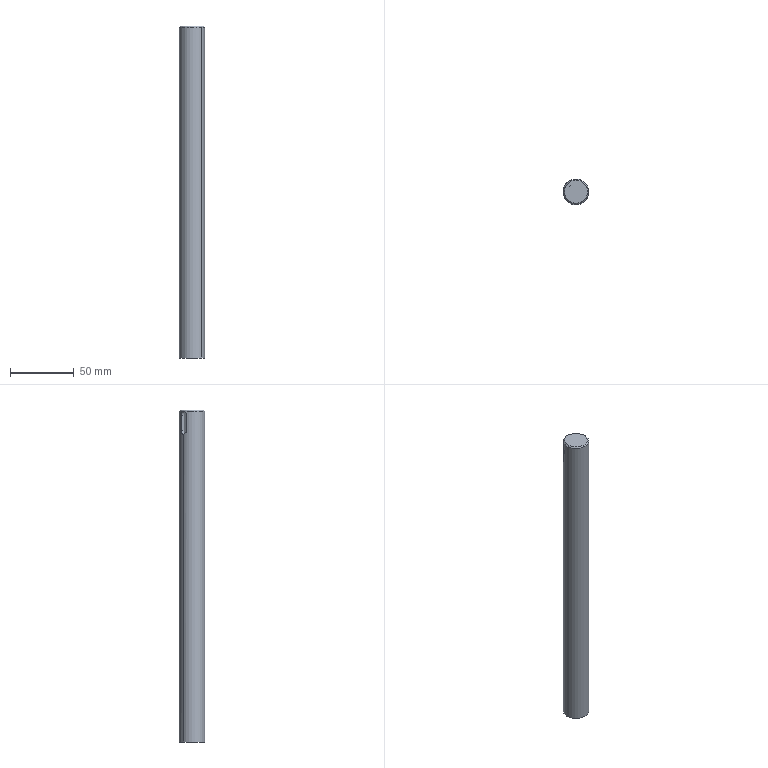Component | SolidWorks | DriveShaft-1 | 1 solid | 11 faces | box 20 x 20 x 260 mm | volume 81314 mm3 | plane 5 | cylinder 4 | cone 2 | commonest cylinder face diameters 20 x2 6 x2
build123d program:
from build123d import *

# Parameters (mm, degrees)
SKETCH1_R           = 10
BOSS_EXTRUDE1_DEPTH = 260
CUT_EXTRUDE1_DEPTH  = 3.5
CHAMFER1_SIZE       = 1


with BuildPart() as part:
    # Sketch1 → Boss-Extrude1 (new body)
    with BuildSketch(Plane(origin=(0, 0, 0), x_dir=(1, 0, 0), z_dir=(0, 1, 0))):
        with Locations(Location((0, 0, 0), (0, 0, 270))):
            Circle(SKETCH1_R)
    extrude(amount=BOSS_EXTRUDE1_DEPTH)

    # Sketch2 → Cut-Extrude1 (cut)
    with BuildSketch(Plane.XY.offset(10)):
        with BuildLine():
            Line((3, 256), (3, 244))
            ThreePointArc((3, 244), (0, 241), (-3, 244))
            Line((-3, 244), (-3, 256))
            ThreePointArc((-3, 256), (0, 259), (3, 256))
        make_face()
    extrude(amount=-CUT_EXTRUDE1_DEPTH, mode=Mode.SUBTRACT)

    # Chamfer1
    chamfer1_edges = [part.edges().sort_by_distance(p)[0] for p in [
        (0, 260, -10),
    ]]
    chamfer(chamfer1_edges, length=CHAMFER1_SIZE)


solid = part.part

# Placed as in the assembly
solid = solid.moved(Location((310.629, 34.1, 218.3), (-90, -48.276, -180)))
STEP:
#1=COLOUR_RGB('',0.7922,0.8196,0.9333);
#2=FILL_AREA_STYLE_COLOUR('',#1);
#3=FILL_AREA_STYLE('',(#2));
#4=SURFACE_STYLE_FILL_AREA(#3);
#5=SURFACE_SIDE_STYLE('',(#4));
#6=SURFACE_STYLE_USAGE(.BOTH.,#5);
#7=PRESENTATION_STYLE_ASSIGNMENT((#6));
#8=CARTESIAN_POINT('',(11.965,1.578,18.831));
#9=VERTEX_POINT('',#8);
#10=CARTESIAN_POINT('',(12.494,1.107,18.831));
#11=VERTEX_POINT('',#10);
#12=CARTESIAN_POINT('',(12.23,1.343,18.831));
#13=DIRECTION('',(0.,0.,1.));
#14=DIRECTION('',(-0.7464,0.6655,0.));
#15=AXIS2_PLACEMENT_3D('',#12,#13,#14);
#16=CIRCLE('',#15,0.3543);
#17=EDGE_CURVE('',#9,#11,#16,.T.);
#18=ORIENTED_EDGE('',*,*,#17,.F.);
#19=CARTESIAN_POINT('',(11.936,1.605,18.791));
#20=VERTEX_POINT('',#19);
#21=CARTESIAN_POINT('',(11.965,1.578,18.831));
#22=DIRECTION('',(-0.5278,0.4706,-0.7071));
#23=VECTOR('',#22,39.37);
#24=LINE('',#21,#23);
#25=EDGE_CURVE('',#9,#20,#24,.T.);
#26=ORIENTED_EDGE('',*,*,#25,.T.);
#27=CARTESIAN_POINT('',(12.523,1.08,18.791));
#28=VERTEX_POINT('',#27);
#29=CARTESIAN_POINT('',(12.23,1.343,18.791));
#30=DIRECTION('',(-0.,-0.,-1.));
#31=DIRECTION('',(-0.7464,0.6655,0.));
#32=AXIS2_PLACEMENT_3D('',#29,#30,#31);
#33=CIRCLE('',#32,0.3937);
#34=EDGE_CURVE('',#28,#20,#33,.T.);
#35=ORIENTED_EDGE('',*,*,#34,.F.);
#36=CARTESIAN_POINT('',(12.494,1.107,18.831));
#37=DIRECTION('',(0.5278,-0.4706,-0.7071));
#38=VECTOR('',#37,39.37);
#39=LINE('',#36,#38);
#40=EDGE_CURVE('',#11,#28,#39,.T.);
#41=ORIENTED_EDGE('',*,*,#40,.F.);
#42=EDGE_LOOP('',(#18,#26,#35,#41));
#43=FACE_OUTER_BOUND('',#42,.T.);
#44=CARTESIAN_POINT('',(12.23,1.343,18.831));
#45=DIRECTION('',(-0.,-0.,-1.));
#46=DIRECTION('',(0.7464,-0.6655,0.));
#47=AXIS2_PLACEMENT_3D('',#44,#45,#46);
#48=CONICAL_SURFACE('',#47,0.3543,0.7854);
#49=ADVANCED_FACE('',(#43),#48,.T.);
#50=CARTESIAN_POINT('',(11.871,1.504,18.201));
#51=VERTEX_POINT('',#50);
#52=CARTESIAN_POINT('',(11.936,1.605,18.083));
#53=VERTEX_POINT('',#52);
#54=CARTESIAN_POINT('',(11.871,1.504,18.201));
#55=CARTESIAN_POINT('',(11.871,1.504,18.193));
#56=CARTESIAN_POINT('',(11.871,1.505,18.185));
#57=CARTESIAN_POINT('',(11.872,1.508,18.17));
#58=CARTESIAN_POINT('',(11.873,1.51,18.163));
#59=CARTESIAN_POINT('',(11.876,1.516,18.148));
#60=CARTESIAN_POINT('',(11.878,1.519,18.141));
#61=CARTESIAN_POINT('',(11.882,1.527,18.129));
#62=CARTESIAN_POINT('',(11.884,1.531,18.123));
#63=CARTESIAN_POINT('',(11.892,1.546,18.106));
#64=CARTESIAN_POINT('',(11.899,1.557,18.098));
#65=CARTESIAN_POINT('',(11.912,1.575,18.089));
#66=CARTESIAN_POINT('',(11.916,1.581,18.086));
#67=CARTESIAN_POINT('',(11.926,1.593,18.083));
#68=CARTESIAN_POINT('',(11.93,1.599,18.083));
#69=CARTESIAN_POINT('',(11.936,1.605,18.083));
#70=B_SPLINE_CURVE_WITH_KNOTS('',3,(#54,#55,#56,#57,#58,#59,#60,#61,#62,#63,#64,#65,#66,#67,#68,#69),.UNSPECIFIED.,.F.,.F.,(4,2,2,2,2,2,2,4),(0.,0.0005898,0.00118,0.001769,0.002359,0.003539,0.004128,0.004718),.UNSPECIFIED.);
#71=EDGE_CURVE('',#51,#53,#70,.T.);
#72=ORIENTED_EDGE('',*,*,#71,.T.);
#73=CARTESIAN_POINT('',(11.936,1.605,8.594));
#74=VERTEX_POINT('',#73);
#75=CARTESIAN_POINT('',(11.936,1.605,18.831));
#76=DIRECTION('',(-0.,-0.,-1.));
#77=VECTOR('',#76,39.37);
#78=LINE('',#75,#77);
#79=EDGE_CURVE('',#53,#74,#78,.T.);
#80=ORIENTED_EDGE('',*,*,#79,.T.);
#81=CARTESIAN_POINT('',(12.523,1.08,8.594));
#82=VERTEX_POINT('',#81);
#83=CARTESIAN_POINT('',(12.23,1.343,8.594));
#84=DIRECTION('',(0.,0.,1.));
#85=DIRECTION('',(-0.7464,0.6655,0.));
#86=AXIS2_PLACEMENT_3D('',#83,#84,#85);
#87=CIRCLE('',#86,0.3937);
#88=EDGE_CURVE('',#74,#82,#87,.T.);
#89=ORIENTED_EDGE('',*,*,#88,.T.);
#90=CARTESIAN_POINT('',(12.523,1.08,18.831));
#91=DIRECTION('',(-0.,-0.,-1.));
#92=VECTOR('',#91,39.37);
#93=LINE('',#90,#92);
#94=EDGE_CURVE('',#28,#82,#93,.T.);
#95=ORIENTED_EDGE('',*,*,#94,.F.);
#96=ORIENTED_EDGE('',*,*,#34,.T.);
#97=CARTESIAN_POINT('',(11.871,1.504,18.673));
#98=VERTEX_POINT('',#97);
#99=CARTESIAN_POINT('',(11.936,1.605,18.791));
#100=CARTESIAN_POINT('',(11.931,1.599,18.791));
#101=CARTESIAN_POINT('',(11.925,1.593,18.791));
#102=CARTESIAN_POINT('',(11.916,1.581,18.788));
#103=CARTESIAN_POINT('',(11.912,1.575,18.785));
#104=CARTESIAN_POINT('',(11.903,1.563,18.779));
#105=CARTESIAN_POINT('',(11.899,1.557,18.776));
#106=CARTESIAN_POINT('',(11.893,1.546,18.767));
#107=CARTESIAN_POINT('',(11.889,1.541,18.762));
#108=CARTESIAN_POINT('',(11.884,1.531,18.751));
#109=CARTESIAN_POINT('',(11.882,1.527,18.745));
#110=CARTESIAN_POINT('',(11.878,1.519,18.733));
#111=CARTESIAN_POINT('',(11.876,1.516,18.726));
#112=CARTESIAN_POINT('',(11.873,1.51,18.712));
#113=CARTESIAN_POINT('',(11.872,1.508,18.704));
#114=CARTESIAN_POINT('',(11.871,1.505,18.689));
#115=CARTESIAN_POINT('',(11.871,1.504,18.681));
#116=CARTESIAN_POINT('',(11.871,1.504,18.673));
#117=B_SPLINE_CURVE_WITH_KNOTS('',3,(#99,#100,#101,#102,#103,#104,#105,#106,#107,#108,#109,#110,#111,#112,#113,#114,#115,#116),.UNSPECIFIED.,.F.,.F.,(4,2,2,2,2,2,2,2,4),(0.004718,0.005307,0.005896,0.006485,0.007074,0.007663,0.008252,0.008842,0.009431),.UNSPECIFIED.);
#118=EDGE_CURVE('',#20,#98,#117,.T.);
#119=ORIENTED_EDGE('',*,*,#118,.T.);
#120=CARTESIAN_POINT('',(11.871,1.504,18.831));
#121=DIRECTION('',(-0.,-0.,-1.));
#122=VECTOR('',#121,39.37);
#123=LINE('',#120,#122);
#124=EDGE_CURVE('',#98,#51,#123,.T.);
#125=ORIENTED_EDGE('',*,*,#124,.T.);
#126=EDGE_LOOP('',(#72,#80,#89,#95,#96,#119,#125));
#127=FACE_OUTER_BOUND('',#126,.T.);
#128=CARTESIAN_POINT('',(12.23,1.343,18.831));
#129=DIRECTION('',(-0.,-0.,-1.));
#130=DIRECTION('',(0.7464,-0.6655,0.));
#131=AXIS2_PLACEMENT_3D('',#128,#129,#130);
#132=CYLINDRICAL_SURFACE('',#131,0.3937);
#133=ADVANCED_FACE('',(#127),#132,.T.);
#134=ORIENTED_EDGE('',*,*,#79,.F.);
#135=CARTESIAN_POINT('',(12.028,1.681,18.201));
#136=VERTEX_POINT('',#135);
#137=CARTESIAN_POINT('',(11.936,1.605,18.083));
#138=CARTESIAN_POINT('',(11.941,1.61,18.083));
#139=CARTESIAN_POINT('',(11.946,1.616,18.083));
#140=CARTESIAN_POINT('',(11.957,1.627,18.086));
#141=CARTESIAN_POINT('',(11.962,1.632,18.089));
#142=CARTESIAN_POINT('',(11.973,1.641,18.095));
#143=CARTESIAN_POINT('',(11.978,1.646,18.098));
#144=CARTESIAN_POINT('',(11.989,1.654,18.107));
#145=CARTESIAN_POINT('',(11.993,1.658,18.112));
#146=CARTESIAN_POINT('',(12.002,1.664,18.123));
#147=CARTESIAN_POINT('',(12.007,1.667,18.129));
#148=CARTESIAN_POINT('',(12.014,1.672,18.141));
#149=CARTESIAN_POINT('',(12.017,1.674,18.148));
#150=CARTESIAN_POINT('',(12.022,1.677,18.163));
#151=CARTESIAN_POINT('',(12.024,1.679,18.17));
#152=CARTESIAN_POINT('',(12.027,1.68,18.185));
#153=CARTESIAN_POINT('',(12.028,1.681,18.193));
#154=CARTESIAN_POINT('',(12.028,1.681,18.201));
#155=B_SPLINE_CURVE_WITH_KNOTS('',3,(#137,#138,#139,#140,#141,#142,#143,#144,#145,#146,#147,#148,#149,#150,#151,#152,#153,#154),.UNSPECIFIED.,.F.,.F.,(4,2,2,2,2,2,2,2,4),(0.004718,0.005307,0.005896,0.006485,0.007074,0.007663,0.008252,0.008842,0.009431),.UNSPECIFIED.);
#156=EDGE_CURVE('',#53,#136,#155,.T.);
#157=ORIENTED_EDGE('',*,*,#156,.T.);
#158=CARTESIAN_POINT('',(12.028,1.681,18.673));
#159=VERTEX_POINT('',#158);
#160=CARTESIAN_POINT('',(12.028,1.681,18.831));
#161=DIRECTION('',(0.,0.,1.));
#162=VECTOR('',#161,39.37);
#163=LINE('',#160,#162);
#164=EDGE_CURVE('',#136,#159,#163,.T.);
#165=ORIENTED_EDGE('',*,*,#164,.T.);
#166=CARTESIAN_POINT('',(12.028,1.681,18.673));
#167=CARTESIAN_POINT('',(12.028,1.681,18.681));
#168=CARTESIAN_POINT('',(12.027,1.68,18.689));
#169=CARTESIAN_POINT('',(12.024,1.679,18.704));
#170=CARTESIAN_POINT('',(12.022,1.677,18.711));
#171=CARTESIAN_POINT('',(12.017,1.674,18.726));
#172=CARTESIAN_POINT('',(12.014,1.672,18.733));
#173=CARTESIAN_POINT('',(12.007,1.667,18.745));
#174=CARTESIAN_POINT('',(12.002,1.664,18.751));
#175=CARTESIAN_POINT('',(11.989,1.654,18.768));
#176=CARTESIAN_POINT('',(11.978,1.646,18.776));
#177=CARTESIAN_POINT('',(11.962,1.632,18.785));
#178=CARTESIAN_POINT('',(11.957,1.627,18.788));
#179=CARTESIAN_POINT('',(11.946,1.616,18.791));
#180=CARTESIAN_POINT('',(11.941,1.61,18.791));
#181=CARTESIAN_POINT('',(11.936,1.605,18.791));
#182=B_SPLINE_CURVE_WITH_KNOTS('',3,(#166,#167,#168,#169,#170,#171,#172,#173,#174,#175,#176,#177,#178,#179,#180,#181),.UNSPECIFIED.,.F.,.F.,(4,2,2,2,2,2,2,4),(0.,0.0005898,0.00118,0.001769,0.002359,0.003539,0.004128,0.004718),.UNSPECIFIED.);
#183=EDGE_CURVE('',#159,#20,#182,.T.);
#184=ORIENTED_EDGE('',*,*,#183,.T.);
#185=CARTESIAN_POINT('',(12.23,1.343,18.791));
#186=DIRECTION('',(-0.,-0.,-1.));
#187=DIRECTION('',(-0.7464,0.6655,0.));
#188=AXIS2_PLACEMENT_3D('',#185,#186,#187);
#189=CIRCLE('',#188,0.3937);
#190=EDGE_CURVE('',#20,#28,#189,.T.);
#191=ORIENTED_EDGE('',*,*,#190,.T.);
#192=ORIENTED_EDGE('',*,*,#94,.T.);
#193=CARTESIAN_POINT('',(12.23,1.343,8.594));
#194=DIRECTION('',(0.,0.,1.));
#195=DIRECTION('',(-0.7464,0.6655,0.));
#196=AXIS2_PLACEMENT_3D('',#193,#194,#195);
#197=CIRCLE('',#196,0.3937);
#198=EDGE_CURVE('',#82,#74,#197,.T.);
#199=ORIENTED_EDGE('',*,*,#198,.T.);
#200=EDGE_LOOP('',(#134,#157,#165,#184,#191,#192,#199));
#201=FACE_OUTER_BOUND('',#200,.T.);
#202=CARTESIAN_POINT('',(12.23,1.343,18.831));
#203=DIRECTION('',(-0.,-0.,-1.));
#204=DIRECTION('',(0.7464,-0.6655,0.));
#205=AXIS2_PLACEMENT_3D('',#202,#203,#204);
#206=CYLINDRICAL_SURFACE('',#205,0.3937);
#207=ADVANCED_FACE('',(#201),#206,.T.);
#208=CARTESIAN_POINT('',(12.23,1.343,18.831));
#209=DIRECTION('',(0.,0.,1.));
#210=DIRECTION('',(-0.7464,0.6655,0.));
#211=AXIS2_PLACEMENT_3D('',#208,#209,#210);
#212=CIRCLE('',#211,0.3543);
#213=EDGE_CURVE('',#11,#9,#212,.T.);
#214=ORIENTED_EDGE('',*,*,#213,.T.);
#215=ORIENTED_EDGE('',*,*,#17,.T.);
#216=EDGE_LOOP('',(#214,#215));
#217=FACE_OUTER_BOUND('',#216,.T.);
#218=CARTESIAN_POINT('',(12.23,1.343,18.831));
#219=DIRECTION('',(0.,0.,1.));
#220=DIRECTION('',(-0.7464,0.6655,0.));
#221=AXIS2_PLACEMENT_3D('',#218,#219,#220);
#222=PLANE('',#221);
#223=ADVANCED_FACE('',(#217),#222,.T.);
#224=ORIENTED_EDGE('',*,*,#198,.F.);
#225=ORIENTED_EDGE('',*,*,#88,.F.);
#226=EDGE_LOOP('',(#224,#225));
#227=FACE_OUTER_BOUND('',#226,.T.);
#228=CARTESIAN_POINT('',(12.23,1.343,8.594));
#229=DIRECTION('',(0.,0.,1.));
#230=DIRECTION('',(-0.7464,0.6655,0.));
#231=AXIS2_PLACEMENT_3D('',#228,#229,#230);
#232=PLANE('',#231);
#233=ADVANCED_FACE('',(#227),#232,.F.);
#234=CARTESIAN_POINT('',(12.117,1.601,18.673));
#235=VERTEX_POINT('',#234);
#236=CARTESIAN_POINT('',(12.117,1.601,18.673));
#237=DIRECTION('',(-0.7464,0.6655,0.));
#238=VECTOR('',#237,39.37);
#239=LINE('',#236,#238);
#240=EDGE_CURVE('',#235,#159,#239,.T.);
#241=ORIENTED_EDGE('',*,*,#240,.F.);
#242=CARTESIAN_POINT('',(11.96,1.425,18.673));
#243=VERTEX_POINT('',#242);
#244=CARTESIAN_POINT('',(12.039,1.513,18.673));
#245=DIRECTION('',(-0.7464,0.6655,0.));
#246=DIRECTION('',(-0.6655,-0.7464,0.));
#247=AXIS2_PLACEMENT_3D('',#244,#245,#246);
#248=CIRCLE('',#247,0.1181);
#249=EDGE_CURVE('',#243,#235,#248,.T.);
#250=ORIENTED_EDGE('',*,*,#249,.F.);
#251=CARTESIAN_POINT('',(11.96,1.425,18.673));
#252=DIRECTION('',(-0.7464,0.6655,0.));
#253=VECTOR('',#252,39.37);
#254=LINE('',#251,#253);
#255=EDGE_CURVE('',#243,#98,#254,.T.);
#256=ORIENTED_EDGE('',*,*,#255,.T.);
#257=ORIENTED_EDGE('',*,*,#118,.F.);
#258=ORIENTED_EDGE('',*,*,#183,.F.);
#259=EDGE_LOOP('',(#241,#250,#256,#257,#258));
#260=FACE_OUTER_BOUND('',#259,.T.);
#261=CARTESIAN_POINT('',(12.039,1.513,18.673));
#262=DIRECTION('',(-0.7464,0.6655,0.));
#263=DIRECTION('',(-0.6655,-0.7464,0.));
#264=AXIS2_PLACEMENT_3D('',#261,#262,#263);
#265=CYLINDRICAL_SURFACE('',#264,0.1181);
#266=ADVANCED_FACE('',(#260),#265,.F.);
#267=ORIENTED_EDGE('',*,*,#255,.F.);
#268=CARTESIAN_POINT('',(11.96,1.425,18.201));
#269=VERTEX_POINT('',#268);
#270=CARTESIAN_POINT('',(11.96,1.425,18.673));
#271=DIRECTION('',(0.,0.,1.));
#272=VECTOR('',#271,39.37);
#273=LINE('',#270,#272);
#274=EDGE_CURVE('',#269,#243,#273,.T.);
#275=ORIENTED_EDGE('',*,*,#274,.F.);
#276=CARTESIAN_POINT('',(11.96,1.425,18.201));
#277=DIRECTION('',(-0.7464,0.6655,0.));
#278=VECTOR('',#277,39.37);
#279=LINE('',#276,#278);
#280=EDGE_CURVE('',#269,#51,#279,.T.);
#281=ORIENTED_EDGE('',*,*,#280,.T.);
#282=ORIENTED_EDGE('',*,*,#124,.F.);
#283=EDGE_LOOP('',(#267,#275,#281,#282));
#284=FACE_OUTER_BOUND('',#283,.T.);
#285=CARTESIAN_POINT('',(11.96,1.425,18.673));
#286=DIRECTION('',(-0.6655,-0.7464,0.));
#287=DIRECTION('',(0.,0.,1.));
#288=AXIS2_PLACEMENT_3D('',#285,#286,#287);
#289=PLANE('',#288);
#290=ADVANCED_FACE('',(#284),#289,.F.);
#291=ORIENTED_EDGE('',*,*,#280,.F.);
#292=CARTESIAN_POINT('',(12.117,1.601,18.201));
#293=VERTEX_POINT('',#292);
#294=CARTESIAN_POINT('',(12.039,1.513,18.201));
#295=DIRECTION('',(-0.7464,0.6655,0.));
#296=DIRECTION('',(-0.6655,-0.7464,0.));
#297=AXIS2_PLACEMENT_3D('',#294,#295,#296);
#298=CIRCLE('',#297,0.1181);
#299=EDGE_CURVE('',#293,#269,#298,.T.);
#300=ORIENTED_EDGE('',*,*,#299,.F.);
#301=CARTESIAN_POINT('',(12.117,1.601,18.201));
#302=DIRECTION('',(-0.7464,0.6655,0.));
#303=VECTOR('',#302,39.37);
#304=LINE('',#301,#303);
#305=EDGE_CURVE('',#293,#136,#304,.T.);
#306=ORIENTED_EDGE('',*,*,#305,.T.);
#307=ORIENTED_EDGE('',*,*,#156,.F.);
#308=ORIENTED_EDGE('',*,*,#71,.F.);
#309=EDGE_LOOP('',(#291,#300,#306,#307,#308));
#310=FACE_OUTER_BOUND('',#309,.T.);
#311=CARTESIAN_POINT('',(12.039,1.513,18.201));
#312=DIRECTION('',(-0.7464,0.6655,0.));
#313=DIRECTION('',(-0.6655,-0.7464,0.));
#314=AXIS2_PLACEMENT_3D('',#311,#312,#313);
#315=CYLINDRICAL_SURFACE('',#314,0.1181);
#316=ADVANCED_FACE('',(#310),#315,.F.);
#317=ORIENTED_EDGE('',*,*,#305,.F.);
#318=CARTESIAN_POINT('',(12.117,1.601,18.673));
#319=DIRECTION('',(-0.,-0.,-1.));
#320=VECTOR('',#319,39.37);
#321=LINE('',#318,#320);
#322=EDGE_CURVE('',#235,#293,#321,.T.);
#323=ORIENTED_EDGE('',*,*,#322,.F.);
#324=ORIENTED_EDGE('',*,*,#240,.T.);
#325=ORIENTED_EDGE('',*,*,#164,.F.);
#326=EDGE_LOOP('',(#317,#323,#324,#325));
#327=FACE_OUTER_BOUND('',#326,.T.);
#328=CARTESIAN_POINT('',(12.117,1.601,18.673));
#329=DIRECTION('',(0.6655,0.7464,-0.));
#330=DIRECTION('',(-0.,-0.,-1.));
#331=AXIS2_PLACEMENT_3D('',#328,#329,#330);
#332=PLANE('',#331);
#333=ADVANCED_FACE('',(#327),#332,.F.);
#334=ORIENTED_EDGE('',*,*,#249,.T.);
#335=ORIENTED_EDGE('',*,*,#322,.T.);
#336=ORIENTED_EDGE('',*,*,#299,.T.);
#337=ORIENTED_EDGE('',*,*,#274,.T.);
#338=EDGE_LOOP('',(#334,#335,#336,#337));
#339=FACE_OUTER_BOUND('',#338,.T.);
#340=CARTESIAN_POINT('',(12.039,1.513,18.673));
#341=DIRECTION('',(-0.7464,0.6655,0.));
#342=DIRECTION('',(-0.6655,-0.7464,0.));
#343=AXIS2_PLACEMENT_3D('',#340,#341,#342);
#344=PLANE('',#343);
#345=ADVANCED_FACE('',(#339),#344,.T.);
#346=ORIENTED_EDGE('',*,*,#25,.F.);
#347=ORIENTED_EDGE('',*,*,#213,.F.);
#348=ORIENTED_EDGE('',*,*,#40,.T.);
#349=ORIENTED_EDGE('',*,*,#190,.F.);
#350=EDGE_LOOP('',(#346,#347,#348,#349));
#351=FACE_OUTER_BOUND('',#350,.T.);
#352=CARTESIAN_POINT('',(12.23,1.343,18.831));
#353=DIRECTION('',(-0.,-0.,-1.));
#354=DIRECTION('',(0.7464,-0.6655,0.));
#355=AXIS2_PLACEMENT_3D('',#352,#353,#354);
#356=CONICAL_SURFACE('',#355,0.3543,0.7854);
#357=ADVANCED_FACE('',(#351),#356,.T.);
#358=CLOSED_SHELL('',(#49,#133,#207,#223,#233,#266,#290,#316,#333,#345,#357));
#359=MANIFOLD_SOLID_BREP('',#358);
#360=STYLED_ITEM('',(#7),#359);
#361=(LENGTH_UNIT()NAMED_UNIT(*)SI_UNIT($,.METRE.));
#362=LENGTH_MEASURE_WITH_UNIT(LENGTH_MEASURE(0.0254),#361);
#363=DIMENSIONAL_EXPONENTS(1.,0.,0.,0.,0.,0.,0.);
#364=(CONVERSION_BASED_UNIT('',#362)LENGTH_UNIT()NAMED_UNIT(#363));
#365=UNCERTAINTY_MEASURE_WITH_UNIT(LENGTH_MEASURE(0.00001),#364,'','');
#366=(NAMED_UNIT(*)PLANE_ANGLE_UNIT()SI_UNIT($,.RADIAN.));
#367=(NAMED_UNIT(*)SI_UNIT($,.STERADIAN.)SOLID_ANGLE_UNIT());
#368=(GEOMETRIC_REPRESENTATION_CONTEXT(3)GLOBAL_UNCERTAINTY_ASSIGNED_CONTEXT((#365))GLOBAL_UNIT_ASSIGNED_CONTEXT((#364,#366,#367))REPRESENTATION_CONTEXT('',''));
#369=MECHANICAL_DESIGN_GEOMETRIC_PRESENTATION_REPRESENTATION('',(#360),#368);
#370=PRESENTATION_LAYER_ASSIGNMENT('','',(#360));
#371=CARTESIAN_POINT('',(0.,0.,0.));
#372=DIRECTION('',(0.,0.,1.));
#373=DIRECTION('',(1.,0.,0.));
#374=AXIS2_PLACEMENT_3D('',#371,#372,#373);
#375=(LENGTH_UNIT()NAMED_UNIT(*)SI_UNIT($,.METRE.));
#376=LENGTH_MEASURE_WITH_UNIT(LENGTH_MEASURE(0.0254),#375);
#377=DIMENSIONAL_EXPONENTS(1.,0.,0.,0.,0.,0.,0.);
#378=(CONVERSION_BASED_UNIT('',#376)LENGTH_UNIT()NAMED_UNIT(#377));
#379=UNCERTAINTY_MEASURE_WITH_UNIT(LENGTH_MEASURE(0.00001),#378,'','');
#380=(NAMED_UNIT(*)PLANE_ANGLE_UNIT()SI_UNIT($,.RADIAN.));
#381=(NAMED_UNIT(*)SI_UNIT($,.STERADIAN.)SOLID_ANGLE_UNIT());
#382=(GEOMETRIC_REPRESENTATION_CONTEXT(3)GLOBAL_UNCERTAINTY_ASSIGNED_CONTEXT((#379))GLOBAL_UNIT_ASSIGNED_CONTEXT((#378,#380,#381))REPRESENTATION_CONTEXT('',''));
#383=ADVANCED_BREP_SHAPE_REPRESENTATION('',(#359,#374),#382);